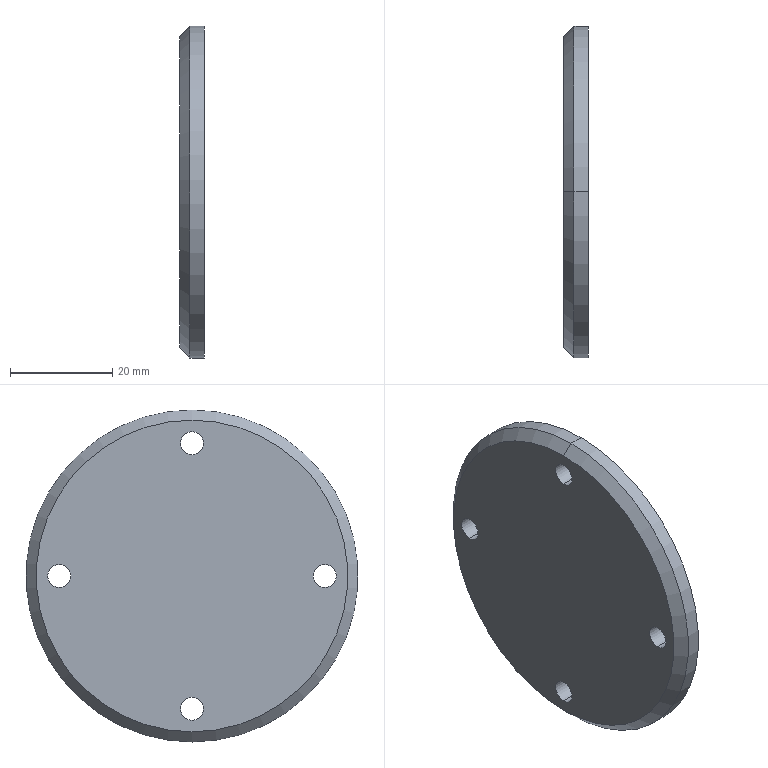Component | SolidWorks | ChainPartBearingOuterEndCap-1 | 1 solid | 17 faces | box 4.8 x 65 x 65 mm | volume 14692 mm3 | cylinder 12 | plane 3 | cone 2 | commonest cylinder face diameters 4.5 x8 26 x2 65 x2
build123d program:
from build123d import *

# Parameters (mm, degrees)
CHAMFER1_SIZE              = 2
F_4_5_4_5_DIAMETER_HOLE1_D = 4.5


with BuildPart() as part:
    # Sketch1 → Revolve1 (revolve)
    with BuildSketch(Plane.XY, mode=Mode.PRIVATE) as revolve1_sk:
        Polygon((0, 0), (32.5, 0), (32.5, 4.8), (13, 4.8), (13, 3.8), (0, 3.8), align=None)
    revolve(revolve1_sk.sketch.rotate(Axis((0, 0, 0), (0, 1, 0)), 90), axis=Axis((0, 0, 0), (0, 1, 0)))

    # Chamfer1
    chamfer1_edges = [part.edges().sort_by_distance(p)[0] for p in [
        (0, 0, 32.5),
    ]]
    chamfer(chamfer1_edges, length=CHAMFER1_SIZE)

    # 4.5 _4.5_ Diameter Hole1 (through all)
    with Locations(Plane(origin=(0, 0, 0), x_dir=(-1, 0, 0), z_dir=(0, -1, 0))):
        with Locations((0, -26), (26, 0), (0, 26), (-26, 0)):
            Hole(F_4_5_4_5_DIAMETER_HOLE1_D / 2)


solid = part.part

# Placed as in the assembly
solid = solid.moved(Location((75.437, -2.563, -35.304), (0, 0, -90)))